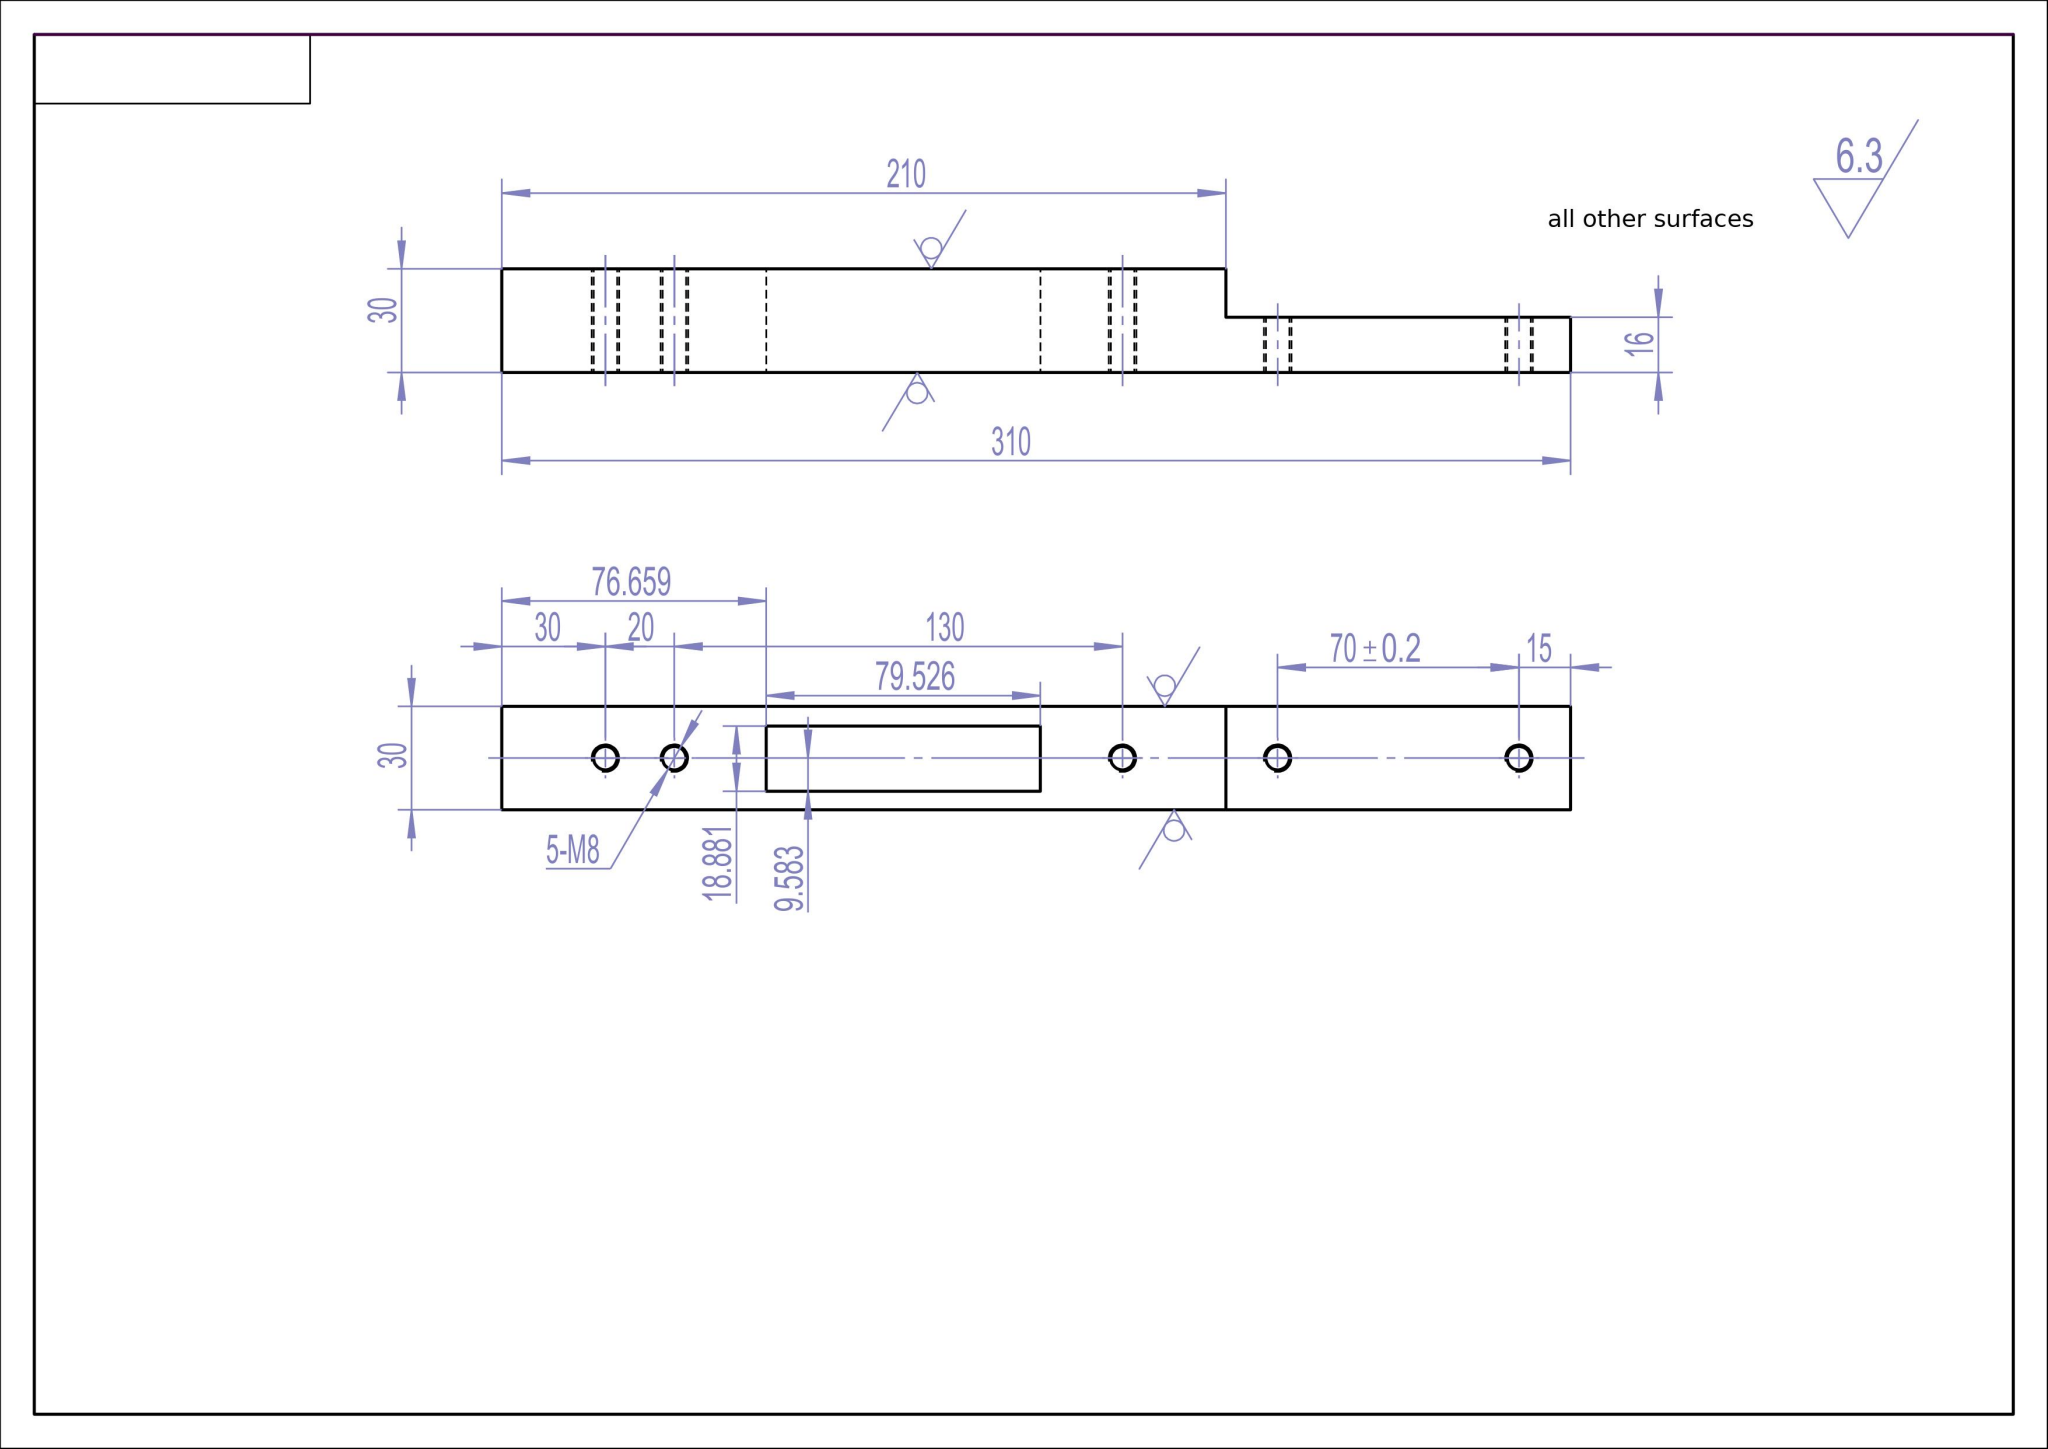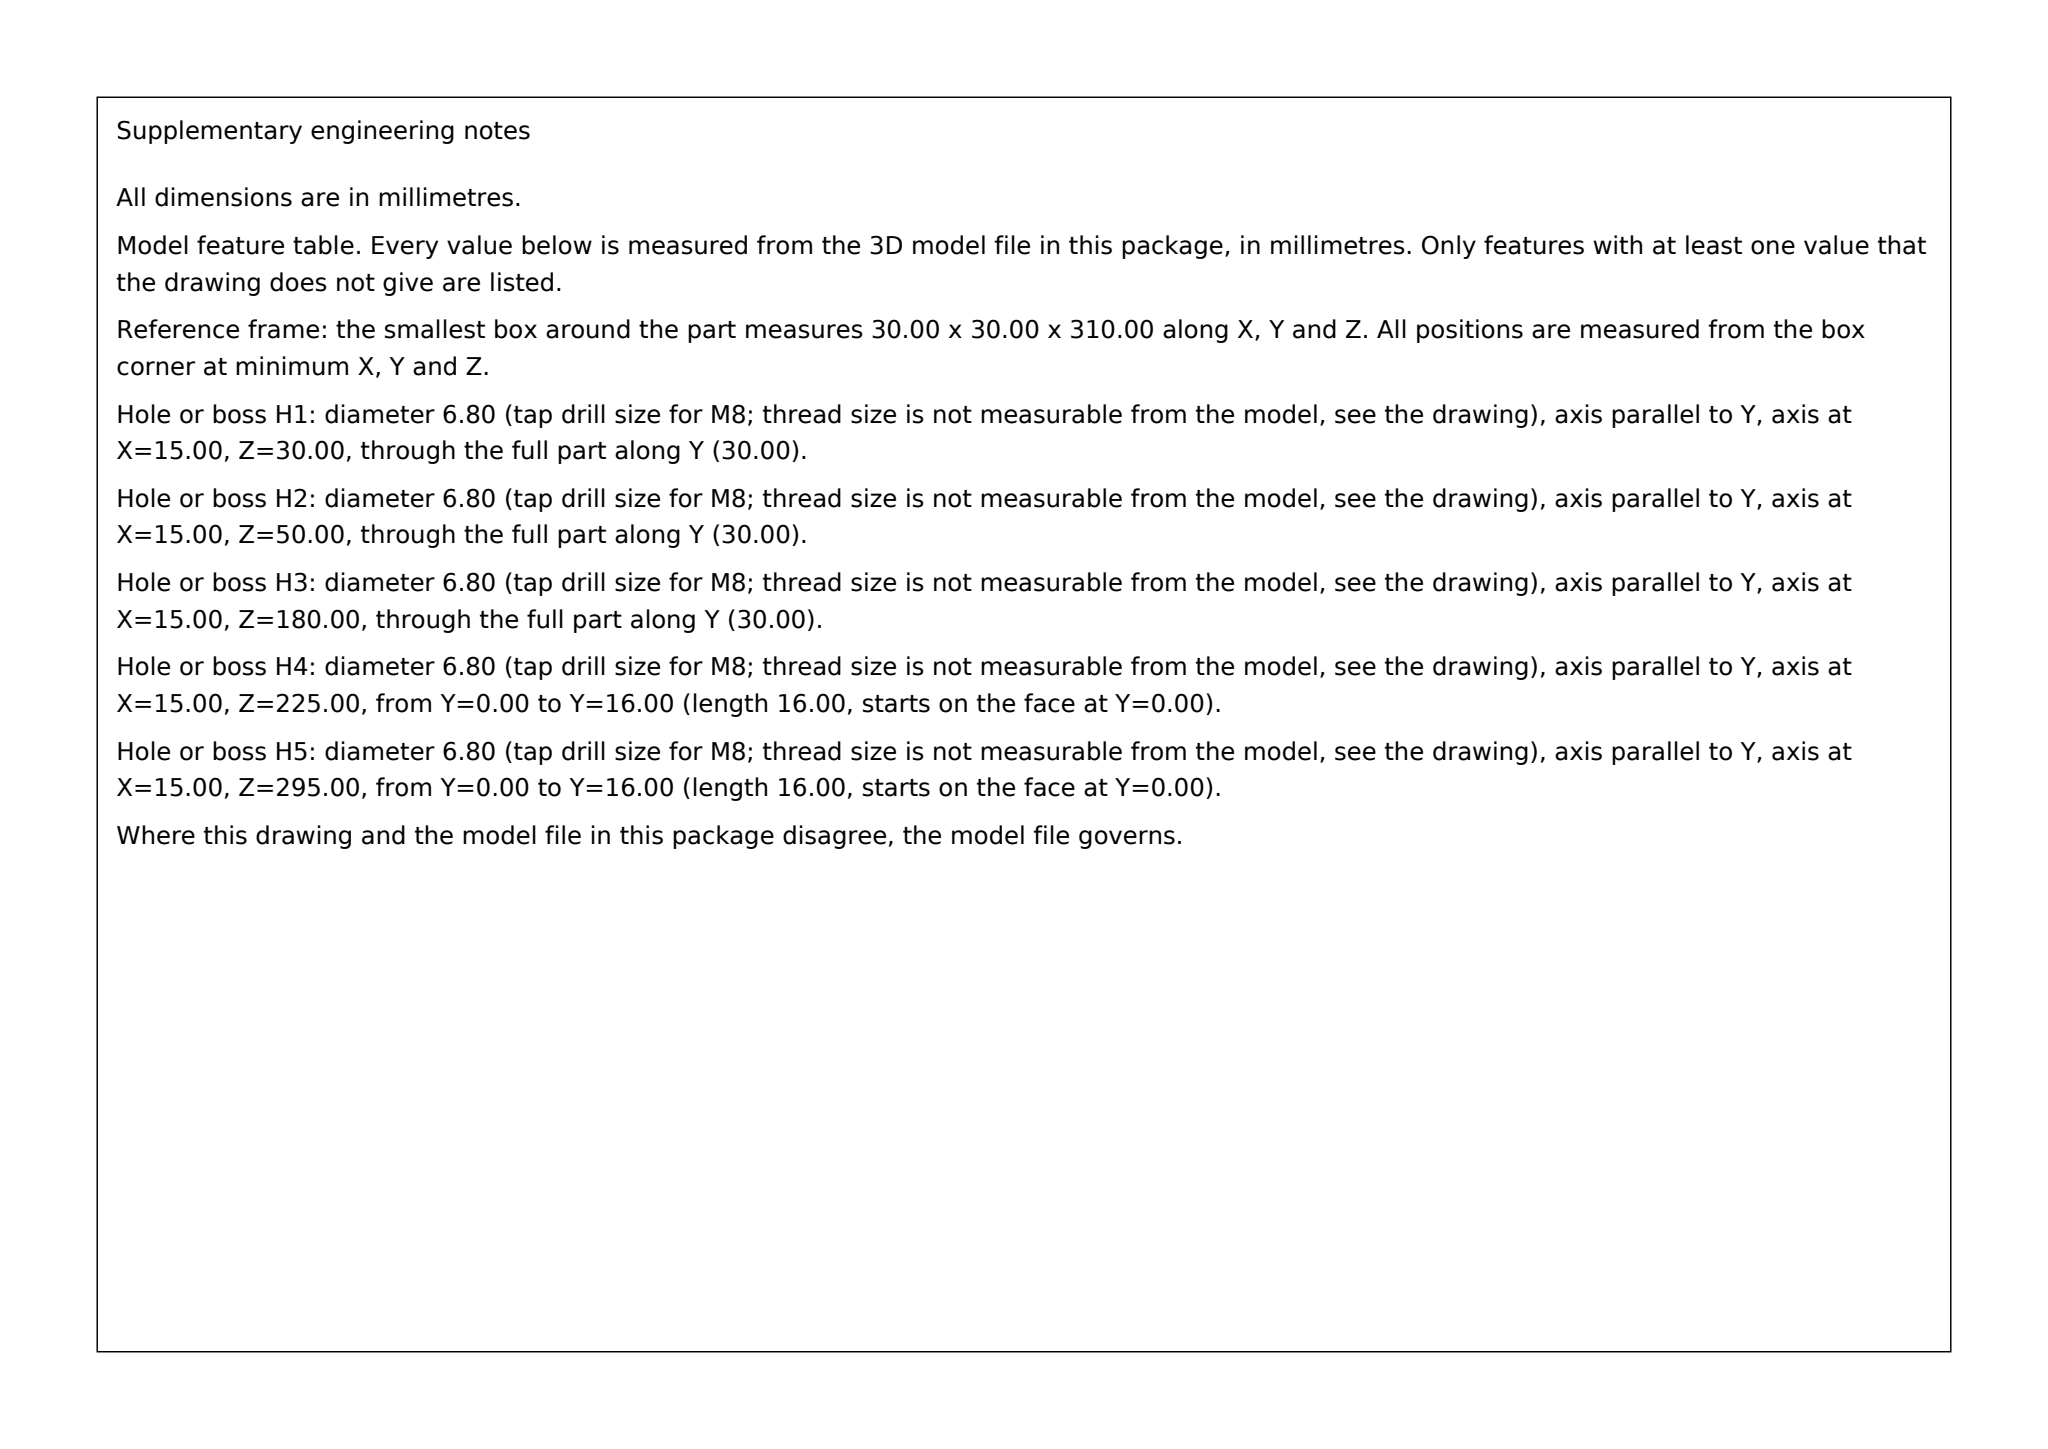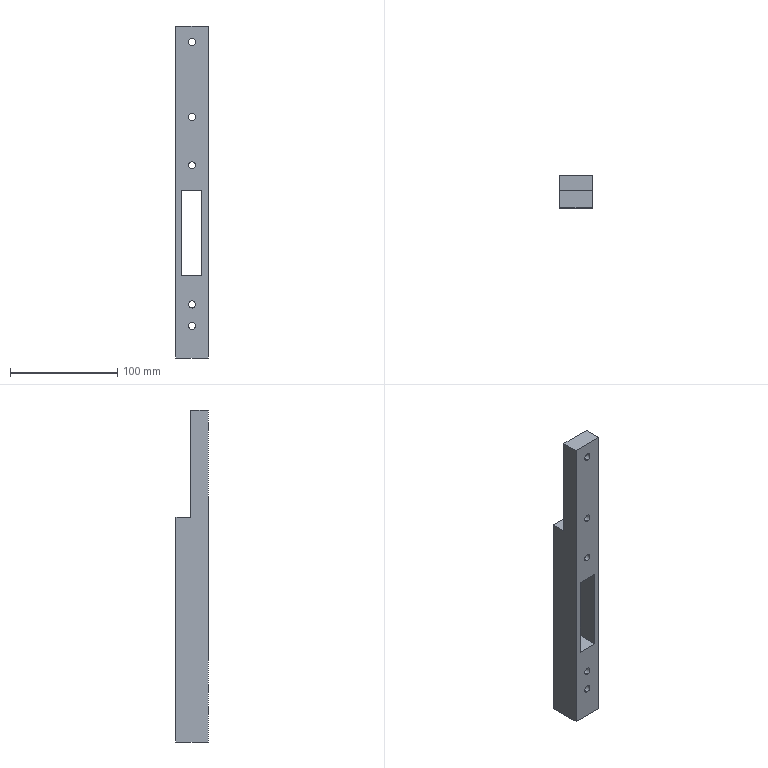Part | SolidWorks | mm | 1 solid | 22 faces | box 30 x 30 x 310 mm | volume 187523 mm3 | plane 12 | cylinder 10 | commonest cylinder face diameters 6.8 x10
build123d program:
from build123d import *

# Parameters (mm, degrees)
SKETCH1_W             = 30
SKETCH1_H             = 30
BOSS_EXTRUDE1_DEPTH   = 310
SKETCH2_W             = 30
SKETCH2_H             = 100
CUT_EXTRUDE1_DEPTH    = 14
M8_TAPPED_HOLE1_D     = 6.8
M8_TAPPED_HOLE1_DEPTH = 39.75
M8_TAPPED_HOLE1_TIP   = 2.043
M8_TAPPED_HOLE2_D     = 6.8
M8_TAPPED_HOLE2_DEPTH = 39.75
M8_TAPPED_HOLE2_TIP   = 2.043
SKETCH7_W             = 18.881
SKETCH7_H             = 79.526
CUT_EXTRUDE2_DEPTH    = 100


with BuildPart() as part:
    # Sketch1 → Boss-Extrude1 (new body)
    with BuildSketch(Plane.XY):
        with Locations((-46.74, 14.494)):
            Rectangle(SKETCH1_W, SKETCH1_H)
    extrude(amount=BOSS_EXTRUDE1_DEPTH)

    # Sketch2 → Cut-Extrude1 (cut)
    with BuildSketch(Plane(origin=(0, 29.494, 0), x_dir=(1, 0, 0), z_dir=(0, 1, 0))):
        with Locations((-46.74, -260)):
            Rectangle(SKETCH2_W, SKETCH2_H)
    extrude(amount=-CUT_EXTRUDE1_DEPTH, mode=Mode.SUBTRACT)

    # M8 Tapped Hole1
    with Locations(Plane(origin=(-46.74, 29.494, 30), x_dir=(0, 0, 1), z_dir=(0, 1, 0))):
        with Locations((0, 0), (20, 0), (150, 0)):
            Hole(M8_TAPPED_HOLE1_D / 2, depth=M8_TAPPED_HOLE1_DEPTH)
            with Locations((0, 0, -(M8_TAPPED_HOLE1_DEPTH + M8_TAPPED_HOLE1_TIP / 2))):  # 118° drill point
                Cone(0, M8_TAPPED_HOLE1_D / 2, M8_TAPPED_HOLE1_TIP, mode=Mode.SUBTRACT)

    # M8 Tapped Hole2
    with Locations(Plane(origin=(-46.74, 15.494, 225), x_dir=(0, 0, 1), z_dir=(0, 1, 0))):
        with Locations((0, 0), (70, 0)):
            Hole(M8_TAPPED_HOLE2_D / 2, depth=M8_TAPPED_HOLE2_DEPTH)
            with Locations((0, 0, -(M8_TAPPED_HOLE2_DEPTH + M8_TAPPED_HOLE2_TIP / 2))):  # 118° drill point
                Cone(0, M8_TAPPED_HOLE2_D / 2, M8_TAPPED_HOLE2_TIP, mode=Mode.SUBTRACT)

    # Sketch7 → Cut-Extrude2 (cut)
    with BuildSketch(Plane(origin=(0, 29.494, 0), x_dir=(1, 0, 0), z_dir=(0, 1, 0))):
        with Locations((-46.882, -116.422)):
            Rectangle(SKETCH7_W, SKETCH7_H)
    extrude(amount=-CUT_EXTRUDE2_DEPTH, mode=Mode.SUBTRACT)


solid = part.part
STEP:
#1=CARTESIAN_POINT('',(-46.74,-0.5058,221.6));
#2=VERTEX_POINT('',#1);
#3=CARTESIAN_POINT('',(-46.74,-0.5058,228.4));
#4=VERTEX_POINT('',#3);
#5=CARTESIAN_POINT('',(-46.74,-0.5058,225.));
#6=DIRECTION('',(0.,1.,0.));
#7=DIRECTION('',(0.,0.,1.));
#8=AXIS2_PLACEMENT_3D('',#5,#6,#7);
#9=CIRCLE('',#8,3.4);
#10=EDGE_CURVE('',#2,#4,#9,.T.);
#11=ORIENTED_EDGE('',*,*,#10,.F.);
#12=CARTESIAN_POINT('',(-46.74,15.494,221.6));
#13=VERTEX_POINT('',#12);
#14=CARTESIAN_POINT('',(-46.74,15.494,221.6));
#15=DIRECTION('',(0.,1.,0.));
#16=VECTOR('',#15,1000.);
#17=LINE('',#14,#16);
#18=EDGE_CURVE('',#2,#13,#17,.T.);
#19=ORIENTED_EDGE('',*,*,#18,.T.);
#20=CARTESIAN_POINT('',(-46.74,15.494,228.4));
#21=VERTEX_POINT('',#20);
#22=CARTESIAN_POINT('',(-46.74,15.494,225.));
#23=DIRECTION('',(0.,1.,0.));
#24=DIRECTION('',(0.,0.,1.));
#25=AXIS2_PLACEMENT_3D('',#22,#23,#24);
#26=CIRCLE('',#25,3.4);
#27=EDGE_CURVE('',#13,#21,#26,.T.);
#28=ORIENTED_EDGE('',*,*,#27,.T.);
#29=CARTESIAN_POINT('',(-46.74,15.494,228.4));
#30=DIRECTION('',(0.,1.,0.));
#31=VECTOR('',#30,1000.);
#32=LINE('',#29,#31);
#33=EDGE_CURVE('',#4,#21,#32,.T.);
#34=ORIENTED_EDGE('',*,*,#33,.F.);
#35=EDGE_LOOP('',(#11,#19,#28,#34));
#36=FACE_OUTER_BOUND('',#35,.T.);
#37=CARTESIAN_POINT('',(-46.74,15.494,225.));
#38=DIRECTION('',(0.,1.,0.));
#39=DIRECTION('',(0.,0.,1.));
#40=AXIS2_PLACEMENT_3D('',#37,#38,#39);
#41=CYLINDRICAL_SURFACE('',#40,3.4);
#42=ADVANCED_FACE('',(#36),#41,.F.);
#43=CARTESIAN_POINT('',(-46.74,-0.5058,291.6));
#44=VERTEX_POINT('',#43);
#45=CARTESIAN_POINT('',(-46.74,-0.5058,298.4));
#46=VERTEX_POINT('',#45);
#47=CARTESIAN_POINT('',(-46.74,-0.5058,295.));
#48=DIRECTION('',(0.,1.,0.));
#49=DIRECTION('',(0.,0.,1.));
#50=AXIS2_PLACEMENT_3D('',#47,#48,#49);
#51=CIRCLE('',#50,3.4);
#52=EDGE_CURVE('',#44,#46,#51,.T.);
#53=ORIENTED_EDGE('',*,*,#52,.F.);
#54=CARTESIAN_POINT('',(-46.74,15.494,291.6));
#55=VERTEX_POINT('',#54);
#56=CARTESIAN_POINT('',(-46.74,15.494,291.6));
#57=DIRECTION('',(0.,1.,0.));
#58=VECTOR('',#57,1000.);
#59=LINE('',#56,#58);
#60=EDGE_CURVE('',#44,#55,#59,.T.);
#61=ORIENTED_EDGE('',*,*,#60,.T.);
#62=CARTESIAN_POINT('',(-46.74,15.494,298.4));
#63=VERTEX_POINT('',#62);
#64=CARTESIAN_POINT('',(-46.74,15.494,295.));
#65=DIRECTION('',(0.,1.,0.));
#66=DIRECTION('',(0.,0.,1.));
#67=AXIS2_PLACEMENT_3D('',#64,#65,#66);
#68=CIRCLE('',#67,3.4);
#69=EDGE_CURVE('',#55,#63,#68,.T.);
#70=ORIENTED_EDGE('',*,*,#69,.T.);
#71=CARTESIAN_POINT('',(-46.74,15.494,298.4));
#72=DIRECTION('',(0.,1.,0.));
#73=VECTOR('',#72,1000.);
#74=LINE('',#71,#73);
#75=EDGE_CURVE('',#46,#63,#74,.T.);
#76=ORIENTED_EDGE('',*,*,#75,.F.);
#77=EDGE_LOOP('',(#53,#61,#70,#76));
#78=FACE_OUTER_BOUND('',#77,.T.);
#79=CARTESIAN_POINT('',(-46.74,15.494,295.));
#80=DIRECTION('',(0.,1.,0.));
#81=DIRECTION('',(0.,0.,1.));
#82=AXIS2_PLACEMENT_3D('',#79,#80,#81);
#83=CYLINDRICAL_SURFACE('',#82,3.4);
#84=ADVANCED_FACE('',(#78),#83,.F.);
#85=CARTESIAN_POINT('',(-46.74,-0.5058,26.6));
#86=VERTEX_POINT('',#85);
#87=CARTESIAN_POINT('',(-46.74,-0.5058,33.4));
#88=VERTEX_POINT('',#87);
#89=CARTESIAN_POINT('',(-46.74,-0.5058,30.));
#90=DIRECTION('',(0.,1.,0.));
#91=DIRECTION('',(0.,0.,1.));
#92=AXIS2_PLACEMENT_3D('',#89,#90,#91);
#93=CIRCLE('',#92,3.4);
#94=EDGE_CURVE('',#86,#88,#93,.T.);
#95=ORIENTED_EDGE('',*,*,#94,.F.);
#96=CARTESIAN_POINT('',(-46.74,29.494,26.6));
#97=VERTEX_POINT('',#96);
#98=CARTESIAN_POINT('',(-46.74,29.494,26.6));
#99=DIRECTION('',(0.,1.,0.));
#100=VECTOR('',#99,1000.);
#101=LINE('',#98,#100);
#102=EDGE_CURVE('',#86,#97,#101,.T.);
#103=ORIENTED_EDGE('',*,*,#102,.T.);
#104=CARTESIAN_POINT('',(-46.74,29.494,33.4));
#105=VERTEX_POINT('',#104);
#106=CARTESIAN_POINT('',(-46.74,29.494,30.));
#107=DIRECTION('',(0.,1.,0.));
#108=DIRECTION('',(0.,0.,1.));
#109=AXIS2_PLACEMENT_3D('',#106,#107,#108);
#110=CIRCLE('',#109,3.4);
#111=EDGE_CURVE('',#97,#105,#110,.T.);
#112=ORIENTED_EDGE('',*,*,#111,.T.);
#113=CARTESIAN_POINT('',(-46.74,29.494,33.4));
#114=DIRECTION('',(0.,1.,0.));
#115=VECTOR('',#114,1000.);
#116=LINE('',#113,#115);
#117=EDGE_CURVE('',#88,#105,#116,.T.);
#118=ORIENTED_EDGE('',*,*,#117,.F.);
#119=EDGE_LOOP('',(#95,#103,#112,#118));
#120=FACE_OUTER_BOUND('',#119,.T.);
#121=CARTESIAN_POINT('',(-46.74,29.494,30.));
#122=DIRECTION('',(0.,1.,0.));
#123=DIRECTION('',(0.,0.,1.));
#124=AXIS2_PLACEMENT_3D('',#121,#122,#123);
#125=CYLINDRICAL_SURFACE('',#124,3.4);
#126=ADVANCED_FACE('',(#120),#125,.F.);
#127=CARTESIAN_POINT('',(-46.74,-0.5058,46.6));
#128=VERTEX_POINT('',#127);
#129=CARTESIAN_POINT('',(-46.74,-0.5058,53.4));
#130=VERTEX_POINT('',#129);
#131=CARTESIAN_POINT('',(-46.74,-0.5058,50.));
#132=DIRECTION('',(0.,1.,0.));
#133=DIRECTION('',(0.,0.,1.));
#134=AXIS2_PLACEMENT_3D('',#131,#132,#133);
#135=CIRCLE('',#134,3.4);
#136=EDGE_CURVE('',#128,#130,#135,.T.);
#137=ORIENTED_EDGE('',*,*,#136,.F.);
#138=CARTESIAN_POINT('',(-46.74,29.494,46.6));
#139=VERTEX_POINT('',#138);
#140=CARTESIAN_POINT('',(-46.74,29.494,46.6));
#141=DIRECTION('',(0.,1.,0.));
#142=VECTOR('',#141,1000.);
#143=LINE('',#140,#142);
#144=EDGE_CURVE('',#128,#139,#143,.T.);
#145=ORIENTED_EDGE('',*,*,#144,.T.);
#146=CARTESIAN_POINT('',(-46.74,29.494,53.4));
#147=VERTEX_POINT('',#146);
#148=CARTESIAN_POINT('',(-46.74,29.494,50.));
#149=DIRECTION('',(0.,1.,0.));
#150=DIRECTION('',(0.,0.,1.));
#151=AXIS2_PLACEMENT_3D('',#148,#149,#150);
#152=CIRCLE('',#151,3.4);
#153=EDGE_CURVE('',#139,#147,#152,.T.);
#154=ORIENTED_EDGE('',*,*,#153,.T.);
#155=CARTESIAN_POINT('',(-46.74,29.494,53.4));
#156=DIRECTION('',(0.,1.,0.));
#157=VECTOR('',#156,1000.);
#158=LINE('',#155,#157);
#159=EDGE_CURVE('',#130,#147,#158,.T.);
#160=ORIENTED_EDGE('',*,*,#159,.F.);
#161=EDGE_LOOP('',(#137,#145,#154,#160));
#162=FACE_OUTER_BOUND('',#161,.T.);
#163=CARTESIAN_POINT('',(-46.74,29.494,50.));
#164=DIRECTION('',(0.,1.,0.));
#165=DIRECTION('',(0.,0.,1.));
#166=AXIS2_PLACEMENT_3D('',#163,#164,#165);
#167=CYLINDRICAL_SURFACE('',#166,3.4);
#168=ADVANCED_FACE('',(#162),#167,.F.);
#169=CARTESIAN_POINT('',(-46.74,-0.5058,176.6));
#170=VERTEX_POINT('',#169);
#171=CARTESIAN_POINT('',(-46.74,-0.5058,183.4));
#172=VERTEX_POINT('',#171);
#173=CARTESIAN_POINT('',(-46.74,-0.5058,180.));
#174=DIRECTION('',(0.,1.,0.));
#175=DIRECTION('',(0.,0.,1.));
#176=AXIS2_PLACEMENT_3D('',#173,#174,#175);
#177=CIRCLE('',#176,3.4);
#178=EDGE_CURVE('',#170,#172,#177,.T.);
#179=ORIENTED_EDGE('',*,*,#178,.F.);
#180=CARTESIAN_POINT('',(-46.74,29.494,176.6));
#181=VERTEX_POINT('',#180);
#182=CARTESIAN_POINT('',(-46.74,29.494,176.6));
#183=DIRECTION('',(0.,1.,0.));
#184=VECTOR('',#183,1000.);
#185=LINE('',#182,#184);
#186=EDGE_CURVE('',#170,#181,#185,.T.);
#187=ORIENTED_EDGE('',*,*,#186,.T.);
#188=CARTESIAN_POINT('',(-46.74,29.494,183.4));
#189=VERTEX_POINT('',#188);
#190=CARTESIAN_POINT('',(-46.74,29.494,180.));
#191=DIRECTION('',(0.,1.,0.));
#192=DIRECTION('',(0.,0.,1.));
#193=AXIS2_PLACEMENT_3D('',#190,#191,#192);
#194=CIRCLE('',#193,3.4);
#195=EDGE_CURVE('',#181,#189,#194,.T.);
#196=ORIENTED_EDGE('',*,*,#195,.T.);
#197=CARTESIAN_POINT('',(-46.74,29.494,183.4));
#198=DIRECTION('',(0.,1.,0.));
#199=VECTOR('',#198,1000.);
#200=LINE('',#197,#199);
#201=EDGE_CURVE('',#172,#189,#200,.T.);
#202=ORIENTED_EDGE('',*,*,#201,.F.);
#203=EDGE_LOOP('',(#179,#187,#196,#202));
#204=FACE_OUTER_BOUND('',#203,.T.);
#205=CARTESIAN_POINT('',(-46.74,29.494,180.));
#206=DIRECTION('',(0.,1.,0.));
#207=DIRECTION('',(0.,0.,1.));
#208=AXIS2_PLACEMENT_3D('',#205,#206,#207);
#209=CYLINDRICAL_SURFACE('',#208,3.4);
#210=ADVANCED_FACE('',(#204),#209,.F.);
#211=CARTESIAN_POINT('',(-61.74,15.494,210.));
#212=VERTEX_POINT('',#211);
#213=CARTESIAN_POINT('',(-61.74,15.494,310.));
#214=VERTEX_POINT('',#213);
#215=CARTESIAN_POINT('',(-61.74,15.494,310.));
#216=DIRECTION('',(0.,0.,1.));
#217=VECTOR('',#216,1000.);
#218=LINE('',#215,#217);
#219=EDGE_CURVE('',#212,#214,#218,.T.);
#220=ORIENTED_EDGE('',*,*,#219,.F.);
#221=CARTESIAN_POINT('',(-61.74,29.494,210.));
#222=VERTEX_POINT('',#221);
#223=CARTESIAN_POINT('',(-61.74,15.494,210.));
#224=DIRECTION('',(0.,1.,0.));
#225=VECTOR('',#224,1000.);
#226=LINE('',#223,#225);
#227=EDGE_CURVE('',#212,#222,#226,.T.);
#228=ORIENTED_EDGE('',*,*,#227,.T.);
#229=CARTESIAN_POINT('',(-61.74,29.494,0.));
#230=VERTEX_POINT('',#229);
#231=CARTESIAN_POINT('',(-61.74,29.494,310.));
#232=DIRECTION('',(0.,0.,-1.));
#233=VECTOR('',#232,1000.);
#234=LINE('',#231,#233);
#235=EDGE_CURVE('',#222,#230,#234,.T.);
#236=ORIENTED_EDGE('',*,*,#235,.T.);
#237=CARTESIAN_POINT('',(-61.74,-0.5058,0.));
#238=VERTEX_POINT('',#237);
#239=CARTESIAN_POINT('',(-61.74,29.494,0.));
#240=DIRECTION('',(0.,-1.,0.));
#241=VECTOR('',#240,1000.);
#242=LINE('',#239,#241);
#243=EDGE_CURVE('',#230,#238,#242,.T.);
#244=ORIENTED_EDGE('',*,*,#243,.T.);
#245=CARTESIAN_POINT('',(-61.74,-0.5058,310.));
#246=VERTEX_POINT('',#245);
#247=CARTESIAN_POINT('',(-61.74,-0.5058,310.));
#248=DIRECTION('',(0.,0.,-1.));
#249=VECTOR('',#248,1000.);
#250=LINE('',#247,#249);
#251=EDGE_CURVE('',#246,#238,#250,.T.);
#252=ORIENTED_EDGE('',*,*,#251,.F.);
#253=CARTESIAN_POINT('',(-61.74,29.494,310.));
#254=DIRECTION('',(0.,-1.,0.));
#255=VECTOR('',#254,1000.);
#256=LINE('',#253,#255);
#257=EDGE_CURVE('',#214,#246,#256,.T.);
#258=ORIENTED_EDGE('',*,*,#257,.F.);
#259=EDGE_LOOP('',(#220,#228,#236,#244,#252,#258));
#260=FACE_OUTER_BOUND('',#259,.T.);
#261=CARTESIAN_POINT('',(-61.74,29.494,310.));
#262=DIRECTION('',(1.,0.,0.));
#263=DIRECTION('',(0.,0.,-1.));
#264=AXIS2_PLACEMENT_3D('',#261,#262,#263);
#265=PLANE('',#264);
#266=ADVANCED_FACE('',(#260),#265,.F.);
#267=CARTESIAN_POINT('',(-37.442,-0.5058,76.659));
#268=VERTEX_POINT('',#267);
#269=CARTESIAN_POINT('',(-56.323,-0.5058,76.659));
#270=VERTEX_POINT('',#269);
#271=CARTESIAN_POINT('',(-61.74,-0.5058,76.659));
#272=DIRECTION('',(-1.,0.,0.));
#273=VECTOR('',#272,1000.);
#274=LINE('',#271,#273);
#275=EDGE_CURVE('',#268,#270,#274,.T.);
#276=ORIENTED_EDGE('',*,*,#275,.T.);
#277=CARTESIAN_POINT('',(-56.323,-0.5058,156.185));
#278=VERTEX_POINT('',#277);
#279=CARTESIAN_POINT('',(-56.323,-0.5058,310.));
#280=DIRECTION('',(0.,0.,1.));
#281=VECTOR('',#280,1000.);
#282=LINE('',#279,#281);
#283=EDGE_CURVE('',#270,#278,#282,.T.);
#284=ORIENTED_EDGE('',*,*,#283,.T.);
#285=CARTESIAN_POINT('',(-37.442,-0.5058,156.185));
#286=VERTEX_POINT('',#285);
#287=CARTESIAN_POINT('',(-61.74,-0.5058,156.185));
#288=DIRECTION('',(1.,0.,0.));
#289=VECTOR('',#288,1000.);
#290=LINE('',#287,#289);
#291=EDGE_CURVE('',#278,#286,#290,.T.);
#292=ORIENTED_EDGE('',*,*,#291,.T.);
#293=CARTESIAN_POINT('',(-37.442,-0.5058,310.));
#294=DIRECTION('',(0.,0.,-1.));
#295=VECTOR('',#294,1000.);
#296=LINE('',#293,#295);
#297=EDGE_CURVE('',#286,#268,#296,.T.);
#298=ORIENTED_EDGE('',*,*,#297,.T.);
#299=EDGE_LOOP('',(#276,#284,#292,#298));
#300=FACE_BOUND('',#299,.T.);
#301=CARTESIAN_POINT('',(-46.74,-0.5058,225.));
#302=DIRECTION('',(0.,1.,0.));
#303=DIRECTION('',(0.,0.,1.));
#304=AXIS2_PLACEMENT_3D('',#301,#302,#303);
#305=CIRCLE('',#304,3.4);
#306=EDGE_CURVE('',#4,#2,#305,.T.);
#307=ORIENTED_EDGE('',*,*,#306,.T.);
#308=ORIENTED_EDGE('',*,*,#10,.T.);
#309=EDGE_LOOP('',(#307,#308));
#310=FACE_BOUND('',#309,.T.);
#311=CARTESIAN_POINT('',(-46.74,-0.5058,295.));
#312=DIRECTION('',(0.,1.,0.));
#313=DIRECTION('',(0.,0.,1.));
#314=AXIS2_PLACEMENT_3D('',#311,#312,#313);
#315=CIRCLE('',#314,3.4);
#316=EDGE_CURVE('',#46,#44,#315,.T.);
#317=ORIENTED_EDGE('',*,*,#316,.T.);
#318=ORIENTED_EDGE('',*,*,#52,.T.);
#319=EDGE_LOOP('',(#317,#318));
#320=FACE_BOUND('',#319,.T.);
#321=CARTESIAN_POINT('',(-46.74,-0.5058,30.));
#322=DIRECTION('',(0.,1.,0.));
#323=DIRECTION('',(0.,0.,1.));
#324=AXIS2_PLACEMENT_3D('',#321,#322,#323);
#325=CIRCLE('',#324,3.4);
#326=EDGE_CURVE('',#88,#86,#325,.T.);
#327=ORIENTED_EDGE('',*,*,#326,.T.);
#328=ORIENTED_EDGE('',*,*,#94,.T.);
#329=EDGE_LOOP('',(#327,#328));
#330=FACE_BOUND('',#329,.T.);
#331=CARTESIAN_POINT('',(-46.74,-0.5058,50.));
#332=DIRECTION('',(0.,1.,0.));
#333=DIRECTION('',(0.,0.,1.));
#334=AXIS2_PLACEMENT_3D('',#331,#332,#333);
#335=CIRCLE('',#334,3.4);
#336=EDGE_CURVE('',#130,#128,#335,.T.);
#337=ORIENTED_EDGE('',*,*,#336,.T.);
#338=ORIENTED_EDGE('',*,*,#136,.T.);
#339=EDGE_LOOP('',(#337,#338));
#340=FACE_BOUND('',#339,.T.);
#341=CARTESIAN_POINT('',(-46.74,-0.5058,180.));
#342=DIRECTION('',(0.,1.,0.));
#343=DIRECTION('',(0.,0.,1.));
#344=AXIS2_PLACEMENT_3D('',#341,#342,#343);
#345=CIRCLE('',#344,3.4);
#346=EDGE_CURVE('',#172,#170,#345,.T.);
#347=ORIENTED_EDGE('',*,*,#346,.T.);
#348=ORIENTED_EDGE('',*,*,#178,.T.);
#349=EDGE_LOOP('',(#347,#348));
#350=FACE_BOUND('',#349,.T.);
#351=CARTESIAN_POINT('',(-31.74,-0.5058,0.));
#352=VERTEX_POINT('',#351);
#353=CARTESIAN_POINT('',(-61.74,-0.5058,0.));
#354=DIRECTION('',(1.,0.,0.));
#355=VECTOR('',#354,1000.);
#356=LINE('',#353,#355);
#357=EDGE_CURVE('',#238,#352,#356,.T.);
#358=ORIENTED_EDGE('',*,*,#357,.T.);
#359=CARTESIAN_POINT('',(-31.74,-0.5058,310.));
#360=VERTEX_POINT('',#359);
#361=CARTESIAN_POINT('',(-31.74,-0.5058,310.));
#362=DIRECTION('',(0.,0.,-1.));
#363=VECTOR('',#362,1000.);
#364=LINE('',#361,#363);
#365=EDGE_CURVE('',#360,#352,#364,.T.);
#366=ORIENTED_EDGE('',*,*,#365,.F.);
#367=CARTESIAN_POINT('',(-61.74,-0.5058,310.));
#368=DIRECTION('',(1.,0.,0.));
#369=VECTOR('',#368,1000.);
#370=LINE('',#367,#369);
#371=EDGE_CURVE('',#246,#360,#370,.T.);
#372=ORIENTED_EDGE('',*,*,#371,.F.);
#373=ORIENTED_EDGE('',*,*,#251,.T.);
#374=EDGE_LOOP('',(#358,#366,#372,#373));
#375=FACE_OUTER_BOUND('',#374,.T.);
#376=CARTESIAN_POINT('',(-61.74,-0.5058,310.));
#377=DIRECTION('',(0.,1.,0.));
#378=DIRECTION('',(0.,0.,1.));
#379=AXIS2_PLACEMENT_3D('',#376,#377,#378);
#380=PLANE('',#379);
#381=ADVANCED_FACE('',(#300,#310,#320,#330,#340,#350,#375),#380,.F.);
#382=CARTESIAN_POINT('',(-31.74,29.494,210.));
#383=VERTEX_POINT('',#382);
#384=CARTESIAN_POINT('',(-31.74,29.494,0.));
#385=VERTEX_POINT('',#384);
#386=CARTESIAN_POINT('',(-31.74,29.494,310.));
#387=DIRECTION('',(0.,0.,-1.));
#388=VECTOR('',#387,1000.);
#389=LINE('',#386,#388);
#390=EDGE_CURVE('',#383,#385,#389,.T.);
#391=ORIENTED_EDGE('',*,*,#390,.F.);
#392=CARTESIAN_POINT('',(-31.74,15.494,210.));
#393=VERTEX_POINT('',#392);
#394=CARTESIAN_POINT('',(-31.74,15.494,210.));
#395=DIRECTION('',(0.,1.,0.));
#396=VECTOR('',#395,1000.);
#397=LINE('',#394,#396);
#398=EDGE_CURVE('',#393,#383,#397,.T.);
#399=ORIENTED_EDGE('',*,*,#398,.F.);
#400=CARTESIAN_POINT('',(-31.74,15.494,310.));
#401=VERTEX_POINT('',#400);
#402=CARTESIAN_POINT('',(-31.74,15.494,310.));
#403=DIRECTION('',(0.,0.,-1.));
#404=VECTOR('',#403,1000.);
#405=LINE('',#402,#404);
#406=EDGE_CURVE('',#401,#393,#405,.T.);
#407=ORIENTED_EDGE('',*,*,#406,.F.);
#408=CARTESIAN_POINT('',(-31.74,29.494,310.));
#409=DIRECTION('',(-0.,1.,0.));
#410=VECTOR('',#409,1000.);
#411=LINE('',#408,#410);
#412=EDGE_CURVE('',#360,#401,#411,.T.);
#413=ORIENTED_EDGE('',*,*,#412,.F.);
#414=ORIENTED_EDGE('',*,*,#365,.T.);
#415=CARTESIAN_POINT('',(-31.74,29.494,0.));
#416=DIRECTION('',(-0.,1.,0.));
#417=VECTOR('',#416,1000.);
#418=LINE('',#415,#417);
#419=EDGE_CURVE('',#352,#385,#418,.T.);
#420=ORIENTED_EDGE('',*,*,#419,.T.);
#421=EDGE_LOOP('',(#391,#399,#407,#413,#414,#420));
#422=FACE_OUTER_BOUND('',#421,.T.);
#423=CARTESIAN_POINT('',(-31.74,29.494,310.));
#424=DIRECTION('',(-1.,-0.,0.));
#425=DIRECTION('',(0.,-1.,0.));
#426=AXIS2_PLACEMENT_3D('',#423,#424,#425);
#427=PLANE('',#426);
#428=ADVANCED_FACE('',(#422),#427,.F.);
#429=CARTESIAN_POINT('',(-56.323,29.494,156.185));
#430=VERTEX_POINT('',#429);
#431=CARTESIAN_POINT('',(-37.442,29.494,156.185));
#432=VERTEX_POINT('',#431);
#433=CARTESIAN_POINT('',(-56.323,29.494,156.185));
#434=DIRECTION('',(1.,0.,0.));
#435=VECTOR('',#434,1000.);
#436=LINE('',#433,#435);
#437=EDGE_CURVE('',#430,#432,#436,.T.);
#438=ORIENTED_EDGE('',*,*,#437,.F.);
#439=CARTESIAN_POINT('',(-56.323,29.494,76.659));
#440=VERTEX_POINT('',#439);
#441=CARTESIAN_POINT('',(-56.323,29.494,76.659));
#442=DIRECTION('',(0.,0.,1.));
#443=VECTOR('',#442,1000.);
#444=LINE('',#441,#443);
#445=EDGE_CURVE('',#440,#430,#444,.T.);
#446=ORIENTED_EDGE('',*,*,#445,.F.);
#447=CARTESIAN_POINT('',(-37.442,29.494,76.659));
#448=VERTEX_POINT('',#447);
#449=CARTESIAN_POINT('',(-56.323,29.494,76.659));
#450=DIRECTION('',(-1.,0.,0.));
#451=VECTOR('',#450,1000.);
#452=LINE('',#449,#451);
#453=EDGE_CURVE('',#448,#440,#452,.T.);
#454=ORIENTED_EDGE('',*,*,#453,.F.);
#455=CARTESIAN_POINT('',(-37.442,29.494,76.659));
#456=DIRECTION('',(0.,0.,-1.));
#457=VECTOR('',#456,1000.);
#458=LINE('',#455,#457);
#459=EDGE_CURVE('',#432,#448,#458,.T.);
#460=ORIENTED_EDGE('',*,*,#459,.F.);
#461=EDGE_LOOP('',(#438,#446,#454,#460));
#462=FACE_BOUND('',#461,.T.);
#463=CARTESIAN_POINT('',(-46.74,29.494,30.));
#464=DIRECTION('',(0.,1.,0.));
#465=DIRECTION('',(0.,0.,1.));
#466=AXIS2_PLACEMENT_3D('',#463,#464,#465);
#467=CIRCLE('',#466,3.4);
#468=EDGE_CURVE('',#105,#97,#467,.T.);
#469=ORIENTED_EDGE('',*,*,#468,.F.);
#470=ORIENTED_EDGE('',*,*,#111,.F.);
#471=EDGE_LOOP('',(#469,#470));
#472=FACE_BOUND('',#471,.T.);
#473=CARTESIAN_POINT('',(-46.74,29.494,50.));
#474=DIRECTION('',(0.,1.,0.));
#475=DIRECTION('',(0.,0.,1.));
#476=AXIS2_PLACEMENT_3D('',#473,#474,#475);
#477=CIRCLE('',#476,3.4);
#478=EDGE_CURVE('',#147,#139,#477,.T.);
#479=ORIENTED_EDGE('',*,*,#478,.F.);
#480=ORIENTED_EDGE('',*,*,#153,.F.);
#481=EDGE_LOOP('',(#479,#480));
#482=FACE_BOUND('',#481,.T.);
#483=CARTESIAN_POINT('',(-46.74,29.494,180.));
#484=DIRECTION('',(0.,1.,0.));
#485=DIRECTION('',(0.,0.,1.));
#486=AXIS2_PLACEMENT_3D('',#483,#484,#485);
#487=CIRCLE('',#486,3.4);
#488=EDGE_CURVE('',#189,#181,#487,.T.);
#489=ORIENTED_EDGE('',*,*,#488,.F.);
#490=ORIENTED_EDGE('',*,*,#195,.F.);
#491=EDGE_LOOP('',(#489,#490));
#492=FACE_BOUND('',#491,.T.);
#493=ORIENTED_EDGE('',*,*,#235,.F.);
#494=CARTESIAN_POINT('',(-61.74,29.494,210.));
#495=DIRECTION('',(-1.,0.,0.));
#496=VECTOR('',#495,1000.);
#497=LINE('',#494,#496);
#498=EDGE_CURVE('',#383,#222,#497,.T.);
#499=ORIENTED_EDGE('',*,*,#498,.F.);
#500=ORIENTED_EDGE('',*,*,#390,.T.);
#501=CARTESIAN_POINT('',(-61.74,29.494,0.));
#502=DIRECTION('',(-1.,0.,0.));
#503=VECTOR('',#502,1000.);
#504=LINE('',#501,#503);
#505=EDGE_CURVE('',#385,#230,#504,.T.);
#506=ORIENTED_EDGE('',*,*,#505,.T.);
#507=EDGE_LOOP('',(#493,#499,#500,#506));
#508=FACE_OUTER_BOUND('',#507,.T.);
#509=CARTESIAN_POINT('',(-61.74,29.494,310.));
#510=DIRECTION('',(0.,-1.,0.));
#511=DIRECTION('',(0.,0.,-1.));
#512=AXIS2_PLACEMENT_3D('',#509,#510,#511);
#513=PLANE('',#512);
#514=ADVANCED_FACE('',(#462,#472,#482,#492,#508),#513,.F.);
#515=CARTESIAN_POINT('',(-61.74,15.494,310.));
#516=DIRECTION('',(1.,0.,0.));
#517=VECTOR('',#516,1000.);
#518=LINE('',#515,#517);
#519=EDGE_CURVE('',#214,#401,#518,.T.);
#520=ORIENTED_EDGE('',*,*,#519,.F.);
#521=ORIENTED_EDGE('',*,*,#257,.T.);
#522=ORIENTED_EDGE('',*,*,#371,.T.);
#523=ORIENTED_EDGE('',*,*,#412,.T.);
#524=EDGE_LOOP('',(#520,#521,#522,#523));
#525=FACE_OUTER_BOUND('',#524,.T.);
#526=CARTESIAN_POINT('',(0.,0.,310.));
#527=DIRECTION('',(0.,0.,1.));
#528=DIRECTION('',(1.,0.,0.));
#529=AXIS2_PLACEMENT_3D('',#526,#527,#528);
#530=PLANE('',#529);
#531=ADVANCED_FACE('',(#525),#530,.T.);
#532=ORIENTED_EDGE('',*,*,#243,.F.);
#533=ORIENTED_EDGE('',*,*,#505,.F.);
#534=ORIENTED_EDGE('',*,*,#419,.F.);
#535=ORIENTED_EDGE('',*,*,#357,.F.);
#536=EDGE_LOOP('',(#532,#533,#534,#535));
#537=FACE_OUTER_BOUND('',#536,.T.);
#538=CARTESIAN_POINT('',(0.,0.,0.));
#539=DIRECTION('',(0.,0.,1.));
#540=DIRECTION('',(1.,0.,0.));
#541=AXIS2_PLACEMENT_3D('',#538,#539,#540);
#542=PLANE('',#541);
#543=ADVANCED_FACE('',(#537),#542,.F.);
#544=ORIENTED_EDGE('',*,*,#498,.T.);
#545=ORIENTED_EDGE('',*,*,#227,.F.);
#546=CARTESIAN_POINT('',(-61.74,15.494,210.));
#547=DIRECTION('',(-1.,0.,0.));
#548=VECTOR('',#547,1000.);
#549=LINE('',#546,#548);
#550=EDGE_CURVE('',#393,#212,#549,.T.);
#551=ORIENTED_EDGE('',*,*,#550,.F.);
#552=ORIENTED_EDGE('',*,*,#398,.T.);
#553=EDGE_LOOP('',(#544,#545,#551,#552));
#554=FACE_OUTER_BOUND('',#553,.T.);
#555=CARTESIAN_POINT('',(-61.74,15.494,210.));
#556=DIRECTION('',(0.,0.,-1.));
#557=DIRECTION('',(-1.,0.,0.));
#558=AXIS2_PLACEMENT_3D('',#555,#556,#557);
#559=PLANE('',#558);
#560=ADVANCED_FACE('',(#554),#559,.F.);
#561=CARTESIAN_POINT('',(-46.74,15.494,225.));
#562=DIRECTION('',(0.,1.,0.));
#563=DIRECTION('',(0.,0.,1.));
#564=AXIS2_PLACEMENT_3D('',#561,#562,#563);
#565=CIRCLE('',#564,3.4);
#566=EDGE_CURVE('',#21,#13,#565,.T.);
#567=ORIENTED_EDGE('',*,*,#566,.F.);
#568=ORIENTED_EDGE('',*,*,#27,.F.);
#569=EDGE_LOOP('',(#567,#568));
#570=FACE_BOUND('',#569,.T.);
#571=CARTESIAN_POINT('',(-46.74,15.494,295.));
#572=DIRECTION('',(0.,1.,0.));
#573=DIRECTION('',(0.,0.,1.));
#574=AXIS2_PLACEMENT_3D('',#571,#572,#573);
#575=CIRCLE('',#574,3.4);
#576=EDGE_CURVE('',#63,#55,#575,.T.);
#577=ORIENTED_EDGE('',*,*,#576,.F.);
#578=ORIENTED_EDGE('',*,*,#69,.F.);
#579=EDGE_LOOP('',(#577,#578));
#580=FACE_BOUND('',#579,.T.);
#581=ORIENTED_EDGE('',*,*,#219,.T.);
#582=ORIENTED_EDGE('',*,*,#519,.T.);
#583=ORIENTED_EDGE('',*,*,#406,.T.);
#584=ORIENTED_EDGE('',*,*,#550,.T.);
#585=EDGE_LOOP('',(#581,#582,#583,#584));
#586=FACE_OUTER_BOUND('',#585,.T.);
#587=CARTESIAN_POINT('',(0.,15.494,0.));
#588=DIRECTION('',(0.,-1.,0.));
#589=DIRECTION('',(0.,0.,-1.));
#590=AXIS2_PLACEMENT_3D('',#587,#588,#589);
#591=PLANE('',#590);
#592=ADVANCED_FACE('',(#570,#580,#586),#591,.F.);
#593=ORIENTED_EDGE('',*,*,#186,.F.);
#594=ORIENTED_EDGE('',*,*,#346,.F.);
#595=ORIENTED_EDGE('',*,*,#201,.T.);
#596=ORIENTED_EDGE('',*,*,#488,.T.);
#597=EDGE_LOOP('',(#593,#594,#595,#596));
#598=FACE_OUTER_BOUND('',#597,.T.);
#599=CARTESIAN_POINT('',(-46.74,29.494,180.));
#600=DIRECTION('',(0.,1.,0.));
#601=DIRECTION('',(0.,0.,1.));
#602=AXIS2_PLACEMENT_3D('',#599,#600,#601);
#603=CYLINDRICAL_SURFACE('',#602,3.4);
#604=ADVANCED_FACE('',(#598),#603,.F.);
#605=ORIENTED_EDGE('',*,*,#144,.F.);
#606=ORIENTED_EDGE('',*,*,#336,.F.);
#607=ORIENTED_EDGE('',*,*,#159,.T.);
#608=ORIENTED_EDGE('',*,*,#478,.T.);
#609=EDGE_LOOP('',(#605,#606,#607,#608));
#610=FACE_OUTER_BOUND('',#609,.T.);
#611=CARTESIAN_POINT('',(-46.74,29.494,50.));
#612=DIRECTION('',(0.,1.,0.));
#613=DIRECTION('',(0.,0.,1.));
#614=AXIS2_PLACEMENT_3D('',#611,#612,#613);
#615=CYLINDRICAL_SURFACE('',#614,3.4);
#616=ADVANCED_FACE('',(#610),#615,.F.);
#617=ORIENTED_EDGE('',*,*,#102,.F.);
#618=ORIENTED_EDGE('',*,*,#326,.F.);
#619=ORIENTED_EDGE('',*,*,#117,.T.);
#620=ORIENTED_EDGE('',*,*,#468,.T.);
#621=EDGE_LOOP('',(#617,#618,#619,#620));
#622=FACE_OUTER_BOUND('',#621,.T.);
#623=CARTESIAN_POINT('',(-46.74,29.494,30.));
#624=DIRECTION('',(0.,1.,0.));
#625=DIRECTION('',(0.,0.,1.));
#626=AXIS2_PLACEMENT_3D('',#623,#624,#625);
#627=CYLINDRICAL_SURFACE('',#626,3.4);
#628=ADVANCED_FACE('',(#622),#627,.F.);
#629=ORIENTED_EDGE('',*,*,#60,.F.);
#630=ORIENTED_EDGE('',*,*,#316,.F.);
#631=ORIENTED_EDGE('',*,*,#75,.T.);
#632=ORIENTED_EDGE('',*,*,#576,.T.);
#633=EDGE_LOOP('',(#629,#630,#631,#632));
#634=FACE_OUTER_BOUND('',#633,.T.);
#635=CARTESIAN_POINT('',(-46.74,15.494,295.));
#636=DIRECTION('',(0.,1.,0.));
#637=DIRECTION('',(0.,0.,1.));
#638=AXIS2_PLACEMENT_3D('',#635,#636,#637);
#639=CYLINDRICAL_SURFACE('',#638,3.4);
#640=ADVANCED_FACE('',(#634),#639,.F.);
#641=ORIENTED_EDGE('',*,*,#18,.F.);
#642=ORIENTED_EDGE('',*,*,#306,.F.);
#643=ORIENTED_EDGE('',*,*,#33,.T.);
#644=ORIENTED_EDGE('',*,*,#566,.T.);
#645=EDGE_LOOP('',(#641,#642,#643,#644));
#646=FACE_OUTER_BOUND('',#645,.T.);
#647=CARTESIAN_POINT('',(-46.74,15.494,225.));
#648=DIRECTION('',(0.,1.,0.));
#649=DIRECTION('',(0.,0.,1.));
#650=AXIS2_PLACEMENT_3D('',#647,#648,#649);
#651=CYLINDRICAL_SURFACE('',#650,3.4);
#652=ADVANCED_FACE('',(#646),#651,.F.);
#653=CARTESIAN_POINT('',(-56.323,-70.506,76.659));
#654=DIRECTION('',(0.,1.,0.));
#655=VECTOR('',#654,1000.);
#656=LINE('',#653,#655);
#657=EDGE_CURVE('',#270,#440,#656,.T.);
#658=ORIENTED_EDGE('',*,*,#657,.T.);
#659=ORIENTED_EDGE('',*,*,#445,.T.);
#660=CARTESIAN_POINT('',(-56.323,-70.506,156.185));
#661=DIRECTION('',(0.,1.,0.));
#662=VECTOR('',#661,1000.);
#663=LINE('',#660,#662);
#664=EDGE_CURVE('',#278,#430,#663,.T.);
#665=ORIENTED_EDGE('',*,*,#664,.F.);
#666=ORIENTED_EDGE('',*,*,#283,.F.);
#667=EDGE_LOOP('',(#658,#659,#665,#666));
#668=FACE_OUTER_BOUND('',#667,.T.);
#669=CARTESIAN_POINT('',(-56.323,-70.506,76.659));
#670=DIRECTION('',(-1.,0.,0.));
#671=DIRECTION('',(0.,0.,1.));
#672=AXIS2_PLACEMENT_3D('',#669,#670,#671);
#673=PLANE('',#672);
#674=ADVANCED_FACE('',(#668),#673,.F.);
#675=CARTESIAN_POINT('',(-37.442,-70.506,76.659));
#676=DIRECTION('',(0.,1.,0.));
#677=VECTOR('',#676,1000.);
#678=LINE('',#675,#677);
#679=EDGE_CURVE('',#268,#448,#678,.T.);
#680=ORIENTED_EDGE('',*,*,#679,.T.);
#681=ORIENTED_EDGE('',*,*,#453,.T.);
#682=ORIENTED_EDGE('',*,*,#657,.F.);
#683=ORIENTED_EDGE('',*,*,#275,.F.);
#684=EDGE_LOOP('',(#680,#681,#682,#683));
#685=FACE_OUTER_BOUND('',#684,.T.);
#686=CARTESIAN_POINT('',(-56.323,-70.506,76.659));
#687=DIRECTION('',(0.,0.,-1.));
#688=DIRECTION('',(-1.,0.,0.));
#689=AXIS2_PLACEMENT_3D('',#686,#687,#688);
#690=PLANE('',#689);
#691=ADVANCED_FACE('',(#685),#690,.F.);
#692=CARTESIAN_POINT('',(-37.442,-70.506,156.185));
#693=DIRECTION('',(0.,1.,0.));
#694=VECTOR('',#693,1000.);
#695=LINE('',#692,#694);
#696=EDGE_CURVE('',#286,#432,#695,.T.);
#697=ORIENTED_EDGE('',*,*,#696,.T.);
#698=ORIENTED_EDGE('',*,*,#459,.T.);
#699=ORIENTED_EDGE('',*,*,#679,.F.);
#700=ORIENTED_EDGE('',*,*,#297,.F.);
#701=EDGE_LOOP('',(#697,#698,#699,#700));
#702=FACE_OUTER_BOUND('',#701,.T.);
#703=CARTESIAN_POINT('',(-37.442,-70.506,76.659));
#704=DIRECTION('',(1.,0.,0.));
#705=DIRECTION('',(0.,0.,-1.));
#706=AXIS2_PLACEMENT_3D('',#703,#704,#705);
#707=PLANE('',#706);
#708=ADVANCED_FACE('',(#702),#707,.F.);
#709=ORIENTED_EDGE('',*,*,#664,.T.);
#710=ORIENTED_EDGE('',*,*,#437,.T.);
#711=ORIENTED_EDGE('',*,*,#696,.F.);
#712=ORIENTED_EDGE('',*,*,#291,.F.);
#713=EDGE_LOOP('',(#709,#710,#711,#712));
#714=FACE_OUTER_BOUND('',#713,.T.);
#715=CARTESIAN_POINT('',(-56.323,-70.506,156.185));
#716=DIRECTION('',(0.,0.,1.));
#717=DIRECTION('',(1.,0.,0.));
#718=AXIS2_PLACEMENT_3D('',#715,#716,#717);
#719=PLANE('',#718);
#720=ADVANCED_FACE('',(#714),#719,.F.);
#721=CLOSED_SHELL('',(#42,#84,#126,#168,#210,#266,#381,#428,#514,#531,#543,#560,#592,#604,#616,#628,#640,#652,#674,#691,#708,#720));
#722=MANIFOLD_SOLID_BREP('',#721);
#723=CARTESIAN_POINT('',(0.,0.,0.));
#724=DIRECTION('',(0.,0.,1.));
#725=DIRECTION('',(1.,0.,0.));
#726=AXIS2_PLACEMENT_3D('',#723,#724,#725);
#727=(LENGTH_UNIT()NAMED_UNIT(*)SI_UNIT(.MILLI.,.METRE.));
#728=UNCERTAINTY_MEASURE_WITH_UNIT(LENGTH_MEASURE(0.00001),#727,'','');
#729=(NAMED_UNIT(*)PLANE_ANGLE_UNIT()SI_UNIT($,.RADIAN.));
#730=(NAMED_UNIT(*)SI_UNIT($,.STERADIAN.)SOLID_ANGLE_UNIT());
#731=(GEOMETRIC_REPRESENTATION_CONTEXT(3)GLOBAL_UNCERTAINTY_ASSIGNED_CONTEXT((#728))GLOBAL_UNIT_ASSIGNED_CONTEXT((#727,#729,#730))REPRESENTATION_CONTEXT('',''));
#732=ADVANCED_BREP_SHAPE_REPRESENTATION('',(#722,#726),#731);